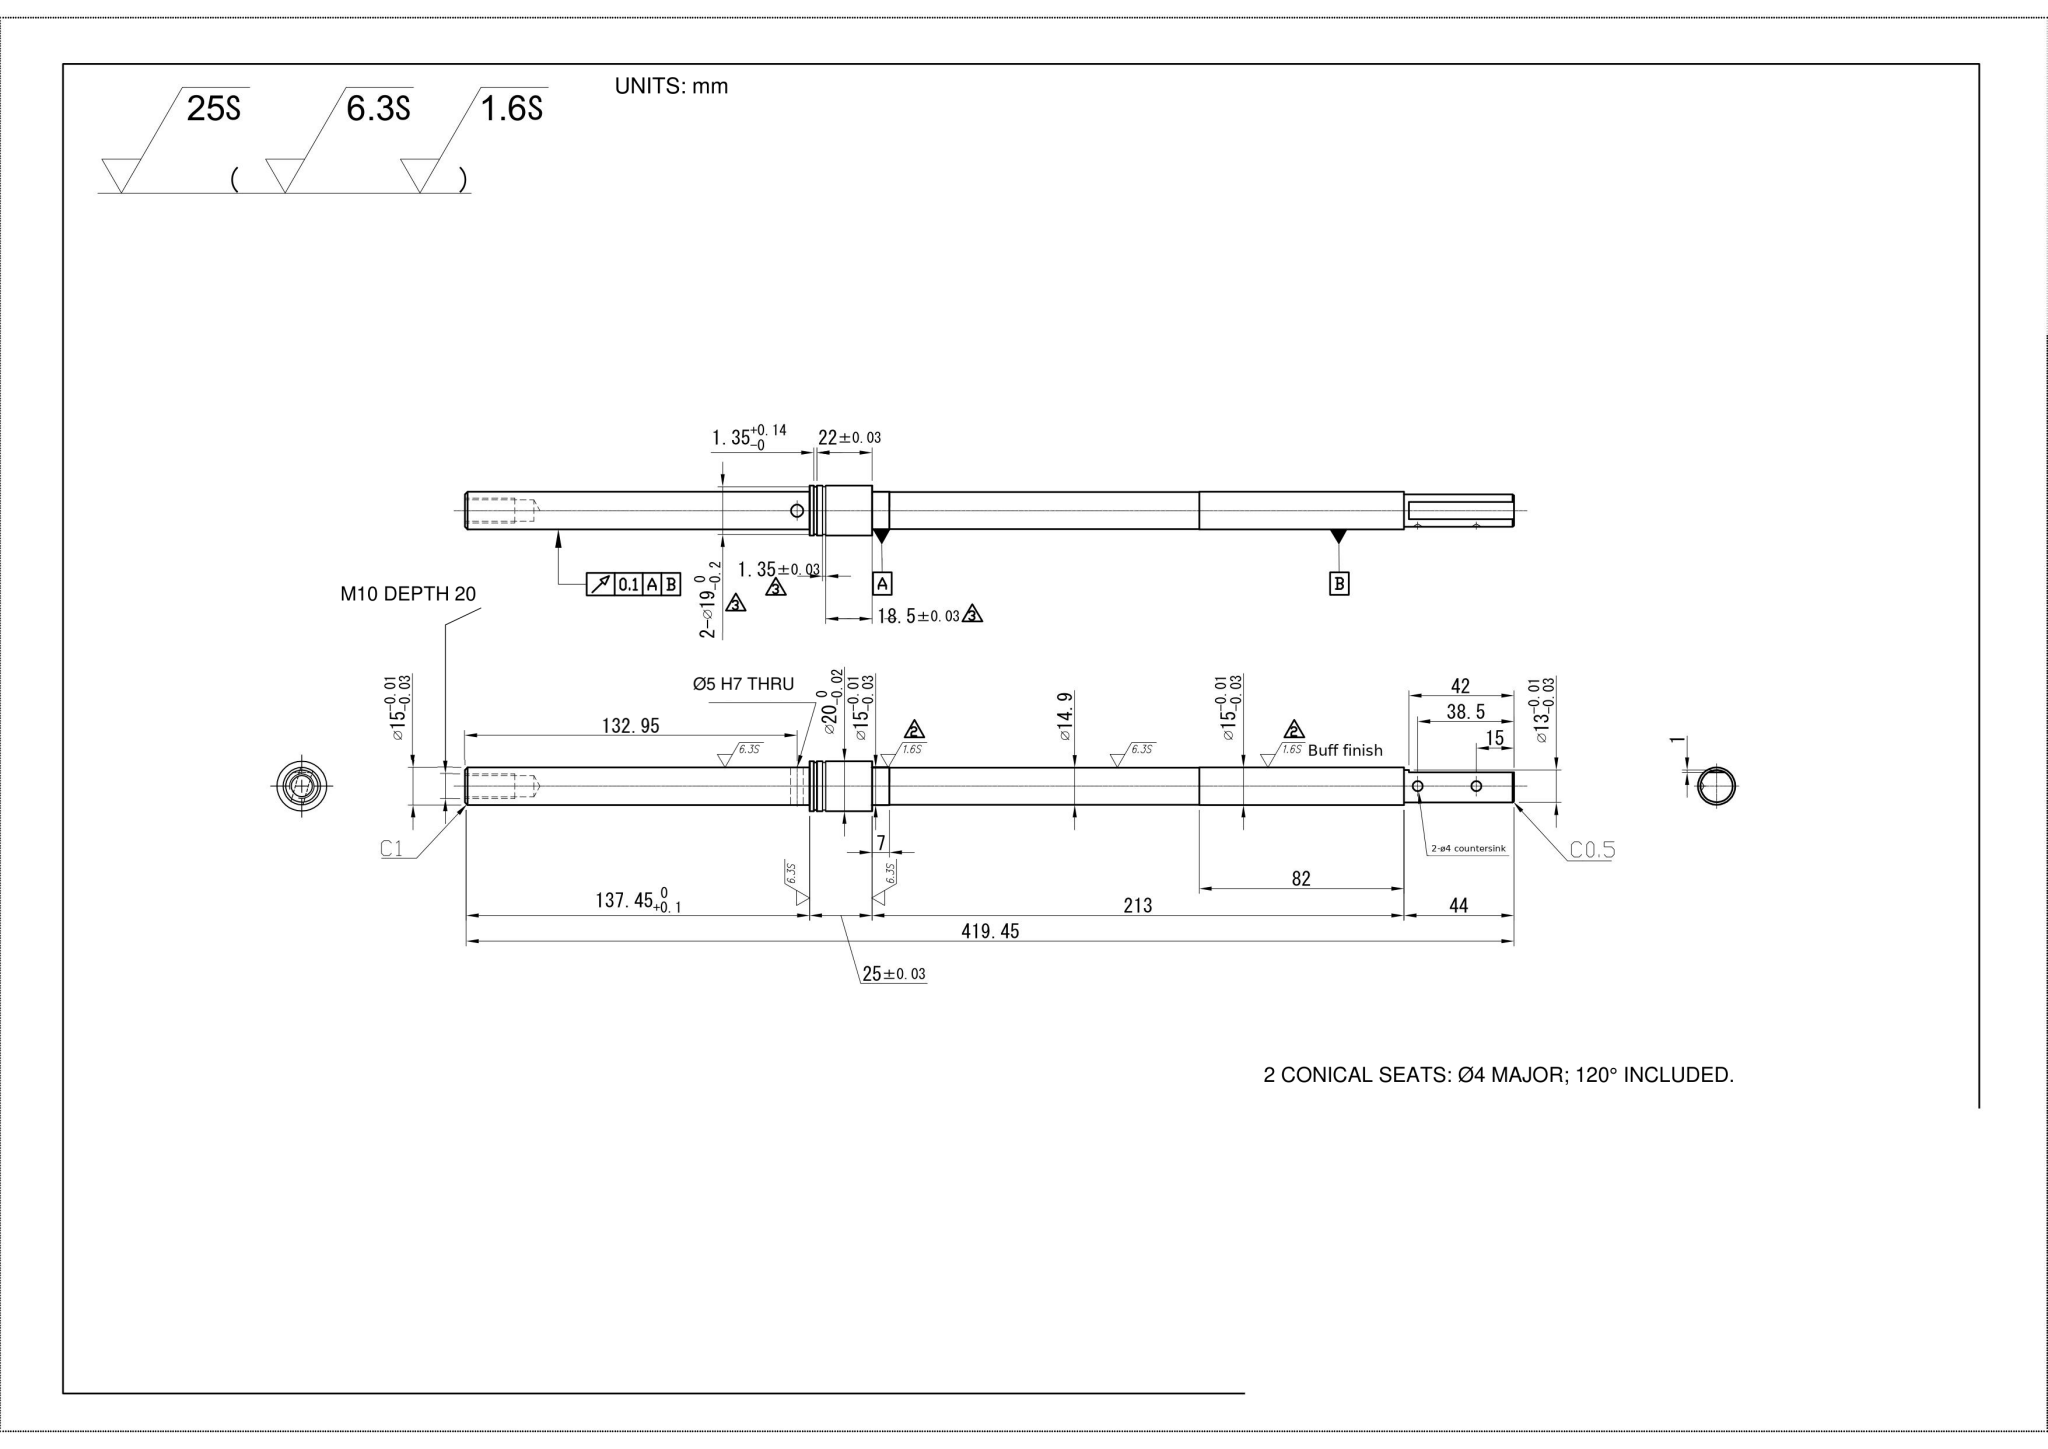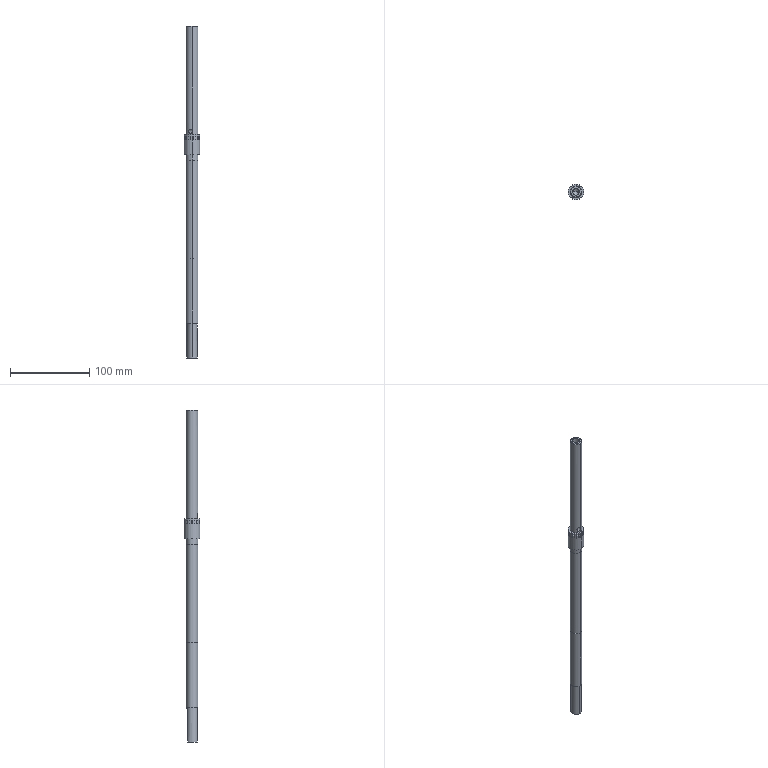Part | NX | mm | 1 solid | 45 faces | box 20 x 20 x 419.45 mm | volume 73123 mm3 | cylinder 24 | plane 13 | cone 8 | commonest cylinder face diameters 20 x6 15 x6 19 x4 14.9 x2 13 x2 5 x2 8.5 x2